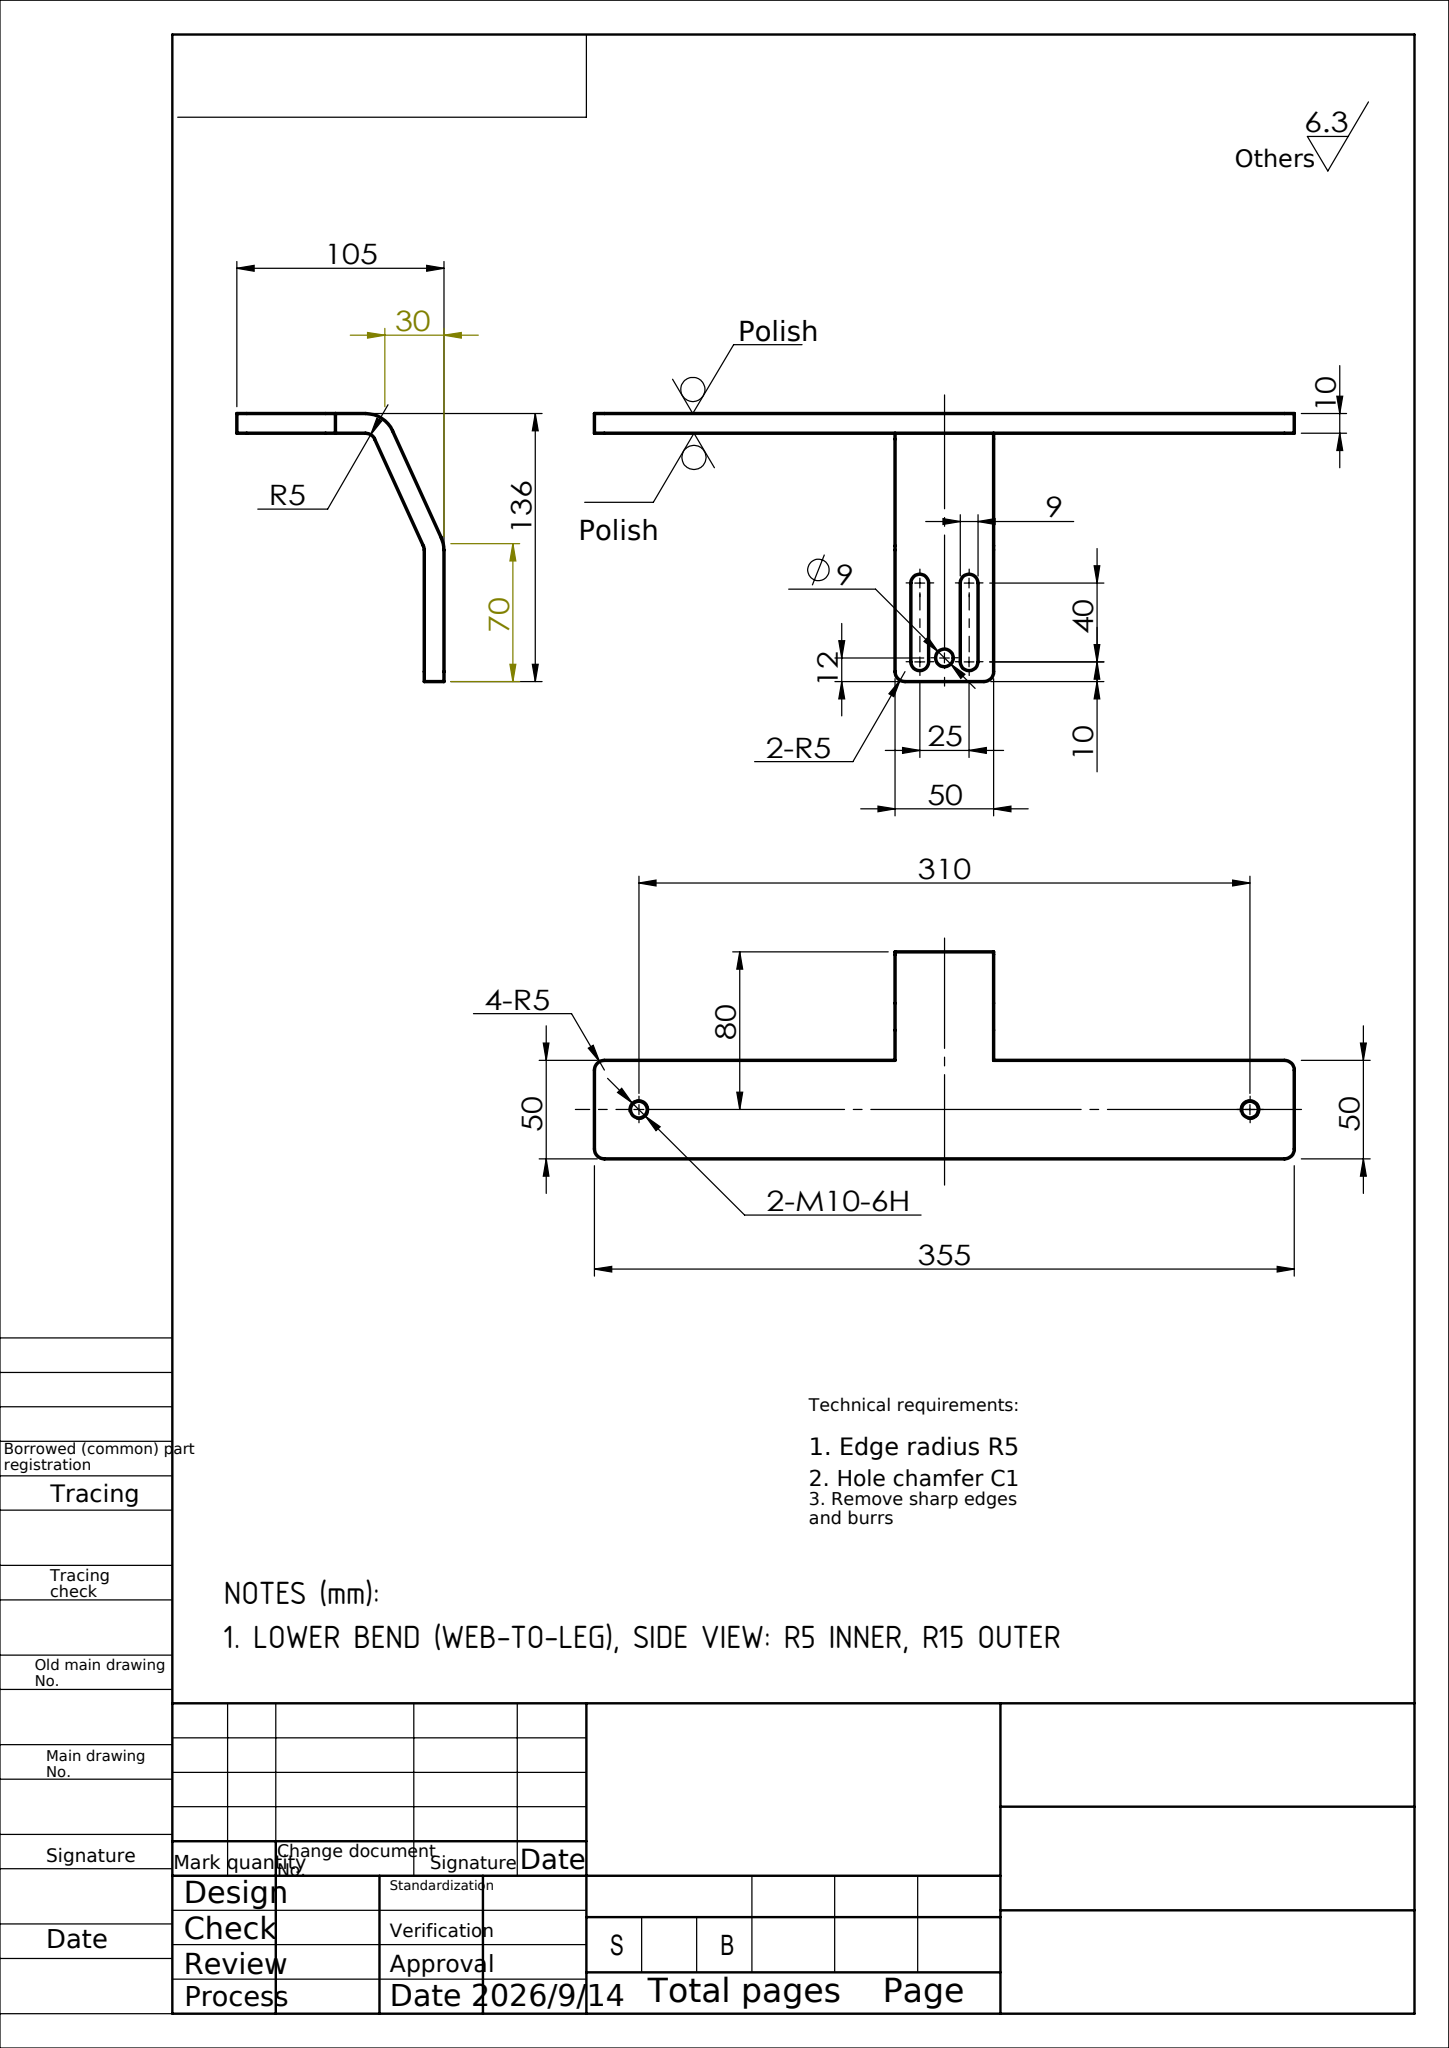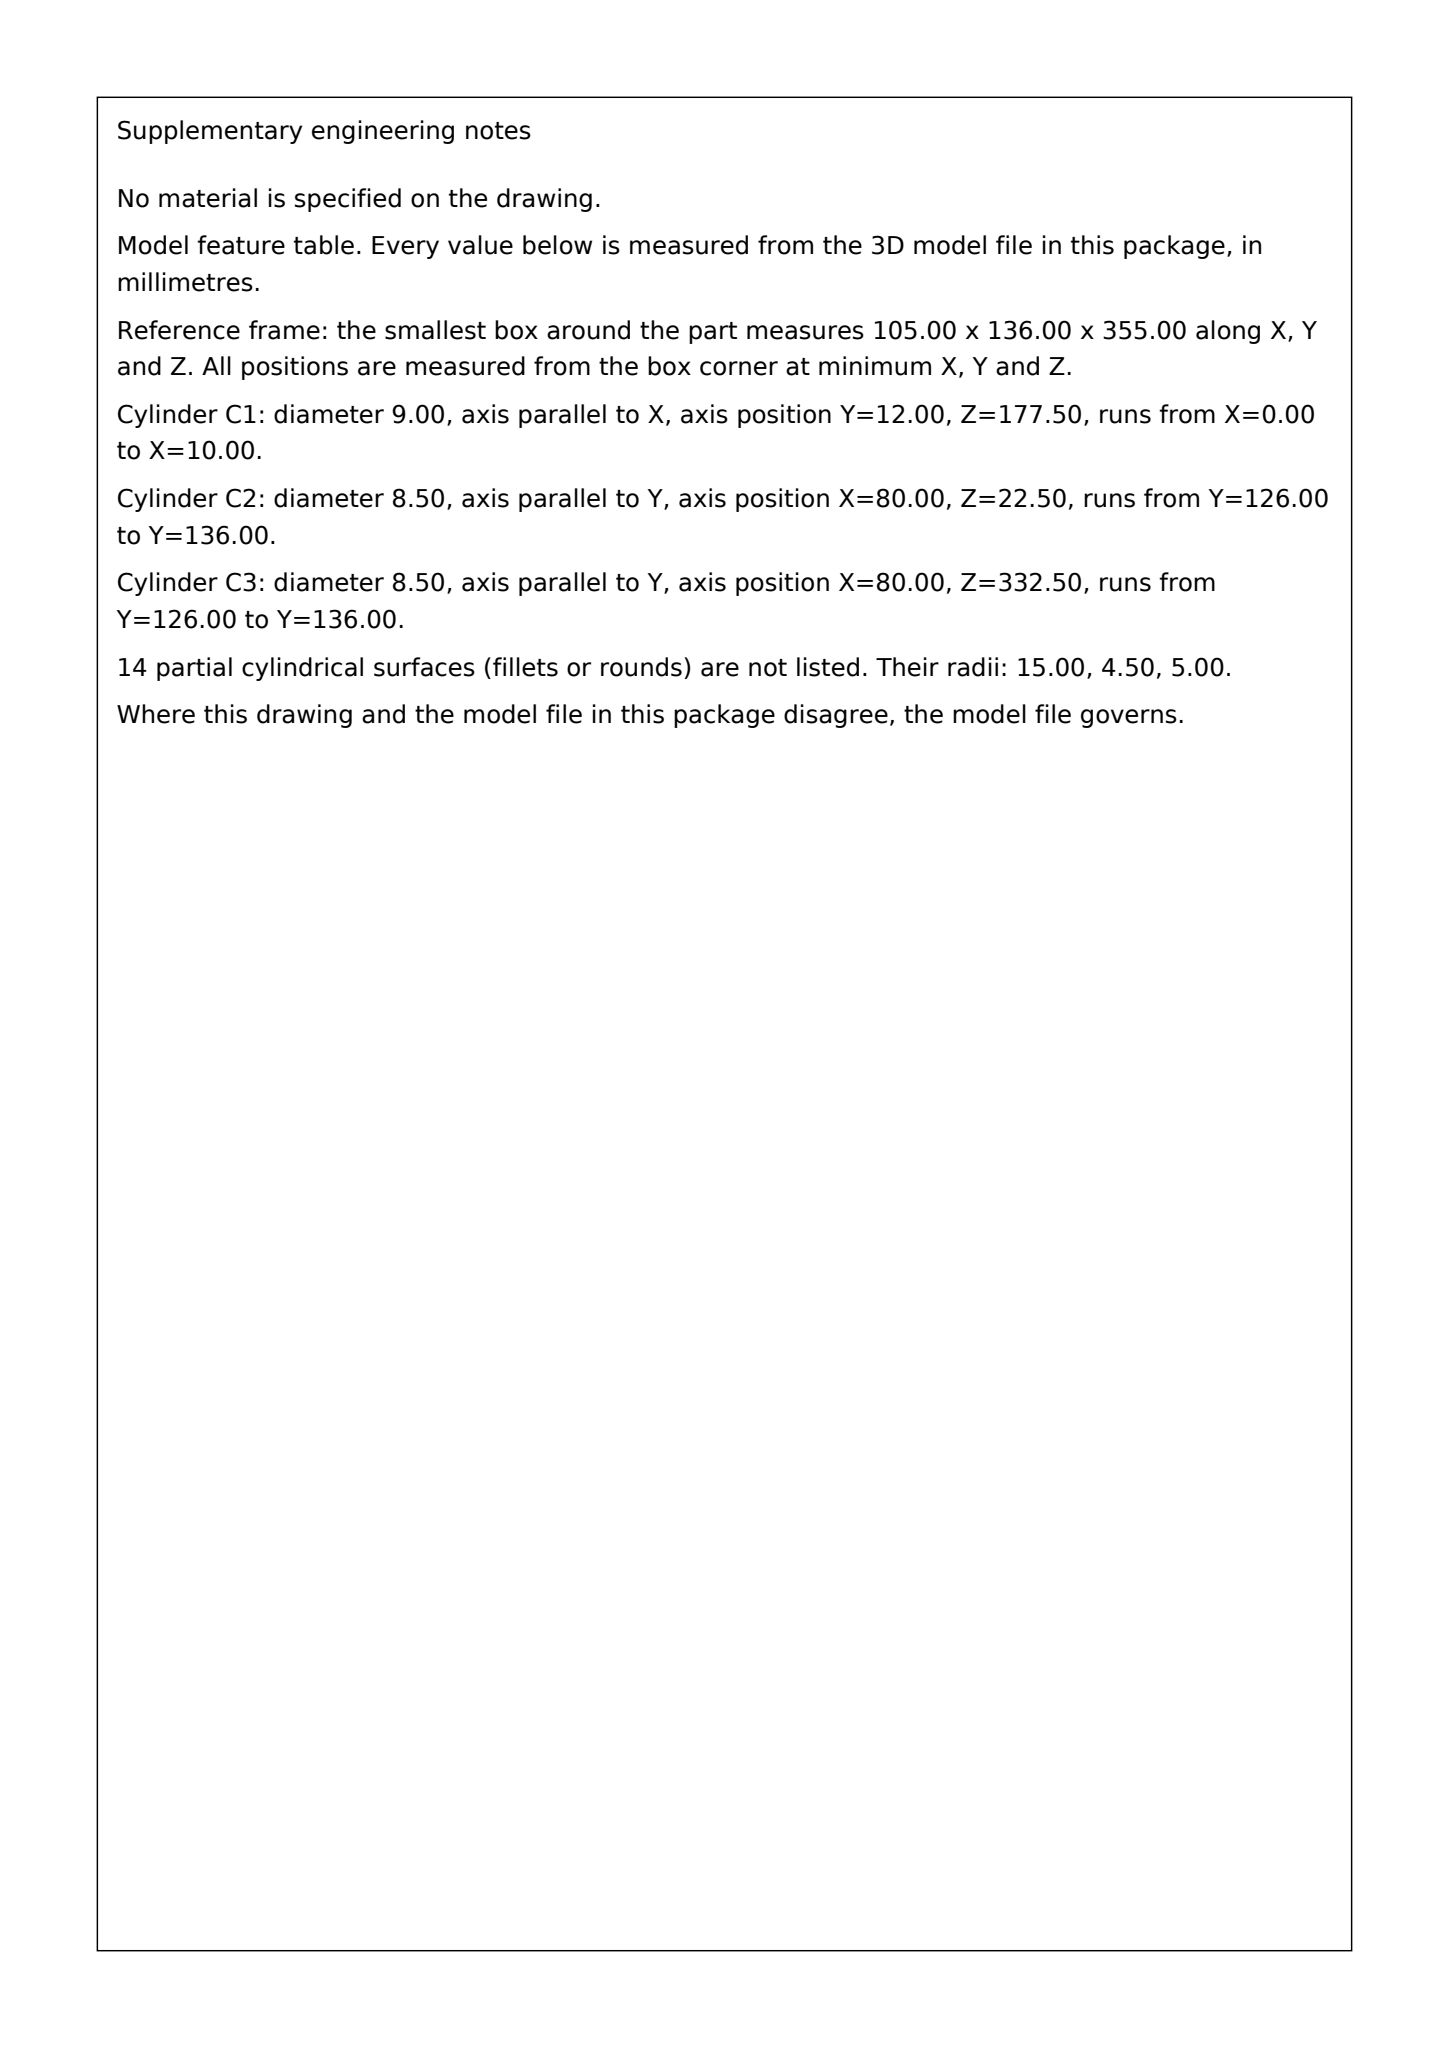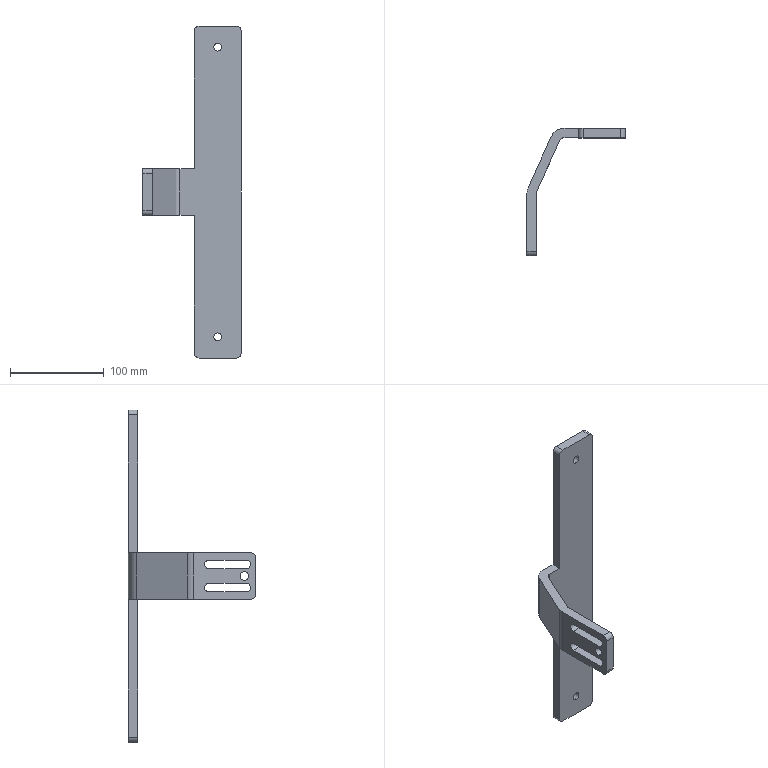Part | SolidWorks | mm | 1 solid | 38 faces | box 105 x 136 x 355 mm | volume 245630 mm3 | cylinder 20 | plane 18 | commonest cylinder face diameters 10 x8 9 x6 8.5 x4 30 x2
Drawing notes:
LOWER BEND (WEB-TO-LEG), SIDE VIEW: R5 INNER, R15 OUTER | from the solid: Z-axis cylinders at (x15.0,y66.75): dia 10.0 (R5 inner) and dia 30.0 (R15 outer), len 50; thk 10
build123d program:
from build123d import *

# Parameters (mm, degrees)
EXTRUDE1_DEPTH     = 25
SKETCH2_W          = 50
SKETCH2_H          = 355
SKETCH2_R          = 3
EXTRUDE2_DEPTH     = 10
M10_TAPPED_HOLE1_D = 8.5
SKETCH5_R          = 4.5
CUT_EXTRUDE1_DEPTH = 10
FILLET1_R          = 5
FILLET2_R          = 15
FILLET3_R          = 5
FILLET4_R          = 15
FILLET5_R          = 5


with BuildPart() as part:
    # Sketch1 → Extrude1 (new, symmetric)
    with BuildSketch(Plane.XY):
        Polygon((0, 0), (0, 70), (30, 136), (55, 136), (55, 126), (36.439, 126), (10, 67.834), (10, 0), align=None)
    extrude(amount=EXTRUDE1_DEPTH, both=True)

    # Sketch2 → Extrude2 (add)
    with BuildSketch(Plane(origin=(0, 136, 0), x_dir=(1, 0, 0), z_dir=(0, 1, 0))):
        with Locations((80, 0)):
            Rectangle(SKETCH2_W, SKETCH2_H)
        with Locations(Location((80, 155, 0), (0, 0, 270))):
            Circle(SKETCH2_R, mode=Mode.SUBTRACT)
        with Locations(Location((80, -155, 0), (0, 0, 270))):
            Circle(SKETCH2_R, mode=Mode.SUBTRACT)
    extrude(amount=-EXTRUDE2_DEPTH)

    # M10 Tapped Hole1 (through all)
    with Locations(Plane(origin=(0, 136, 0), x_dir=(-1, 0, 0), z_dir=(0, 1, 0))):
        with Locations((-80, -155), (-80, 155)):
            Hole(M10_TAPPED_HOLE1_D / 2)

    # Sketch5 → Cut-Extrude1 (cut)
    with BuildSketch(Plane(origin=(10, 0, 0), x_dir=(0, 0, -1), z_dir=(1, 0, 0))):
        with Locations((0, 12)):
            Circle(SKETCH5_R)
        with BuildLine():
            Line((-17, 50), (-17, 10))
            ThreePointArc((-17, 10), (-12.5, 5.5), (-8, 10))
            Line((-8, 10), (-8, 50))
            ThreePointArc((-8, 50), (-12.5, 54.5), (-17, 50))
        make_face()
        with BuildLine():
            Line((8, 10), (8, 50))
            ThreePointArc((8, 50), (12.5, 54.5), (17, 50))
            Line((17, 50), (17, 10))
            ThreePointArc((17, 10), (12.5, 5.5), (8, 10))
        make_face()
    extrude(amount=-CUT_EXTRUDE1_DEPTH, mode=Mode.SUBTRACT)

    # Fillet1
    fillet1_edges = [part.edges().sort_by_distance(p)[0] for p in [
        (5, 0, -25),
        (5, 0, 25),
        (105, 131, 177.5),
        (55, 131, 177.5),
        (55, 131, -177.5),
        (105, 131, -177.5),
    ]]
    fillet(fillet1_edges, radius=FILLET1_R)

    # Fillet2
    fillet2_edges = [part.edges().sort_by_distance(p)[0] for p in [
        (30, 136, 0),
    ]]
    fillet(fillet2_edges, radius=FILLET2_R)

    # Fillet3
    fillet3_edges = [part.edges().sort_by_distance(p)[0] for p in [
        (36.439, 126, 0),
    ]]
    fillet(fillet3_edges, radius=FILLET3_R)

    # Fillet4
    fillet4_edges = [part.edges().sort_by_distance(p)[0] for p in [
        (0, 70, 0),
    ]]
    fillet(fillet4_edges, radius=FILLET4_R)

    # Fillet5
    fillet5_edges = [part.edges().sort_by_distance(p)[0] for p in [
        (10, 67.834, 0),
    ]]
    fillet(fillet5_edges, radius=FILLET5_R)


solid = part.part